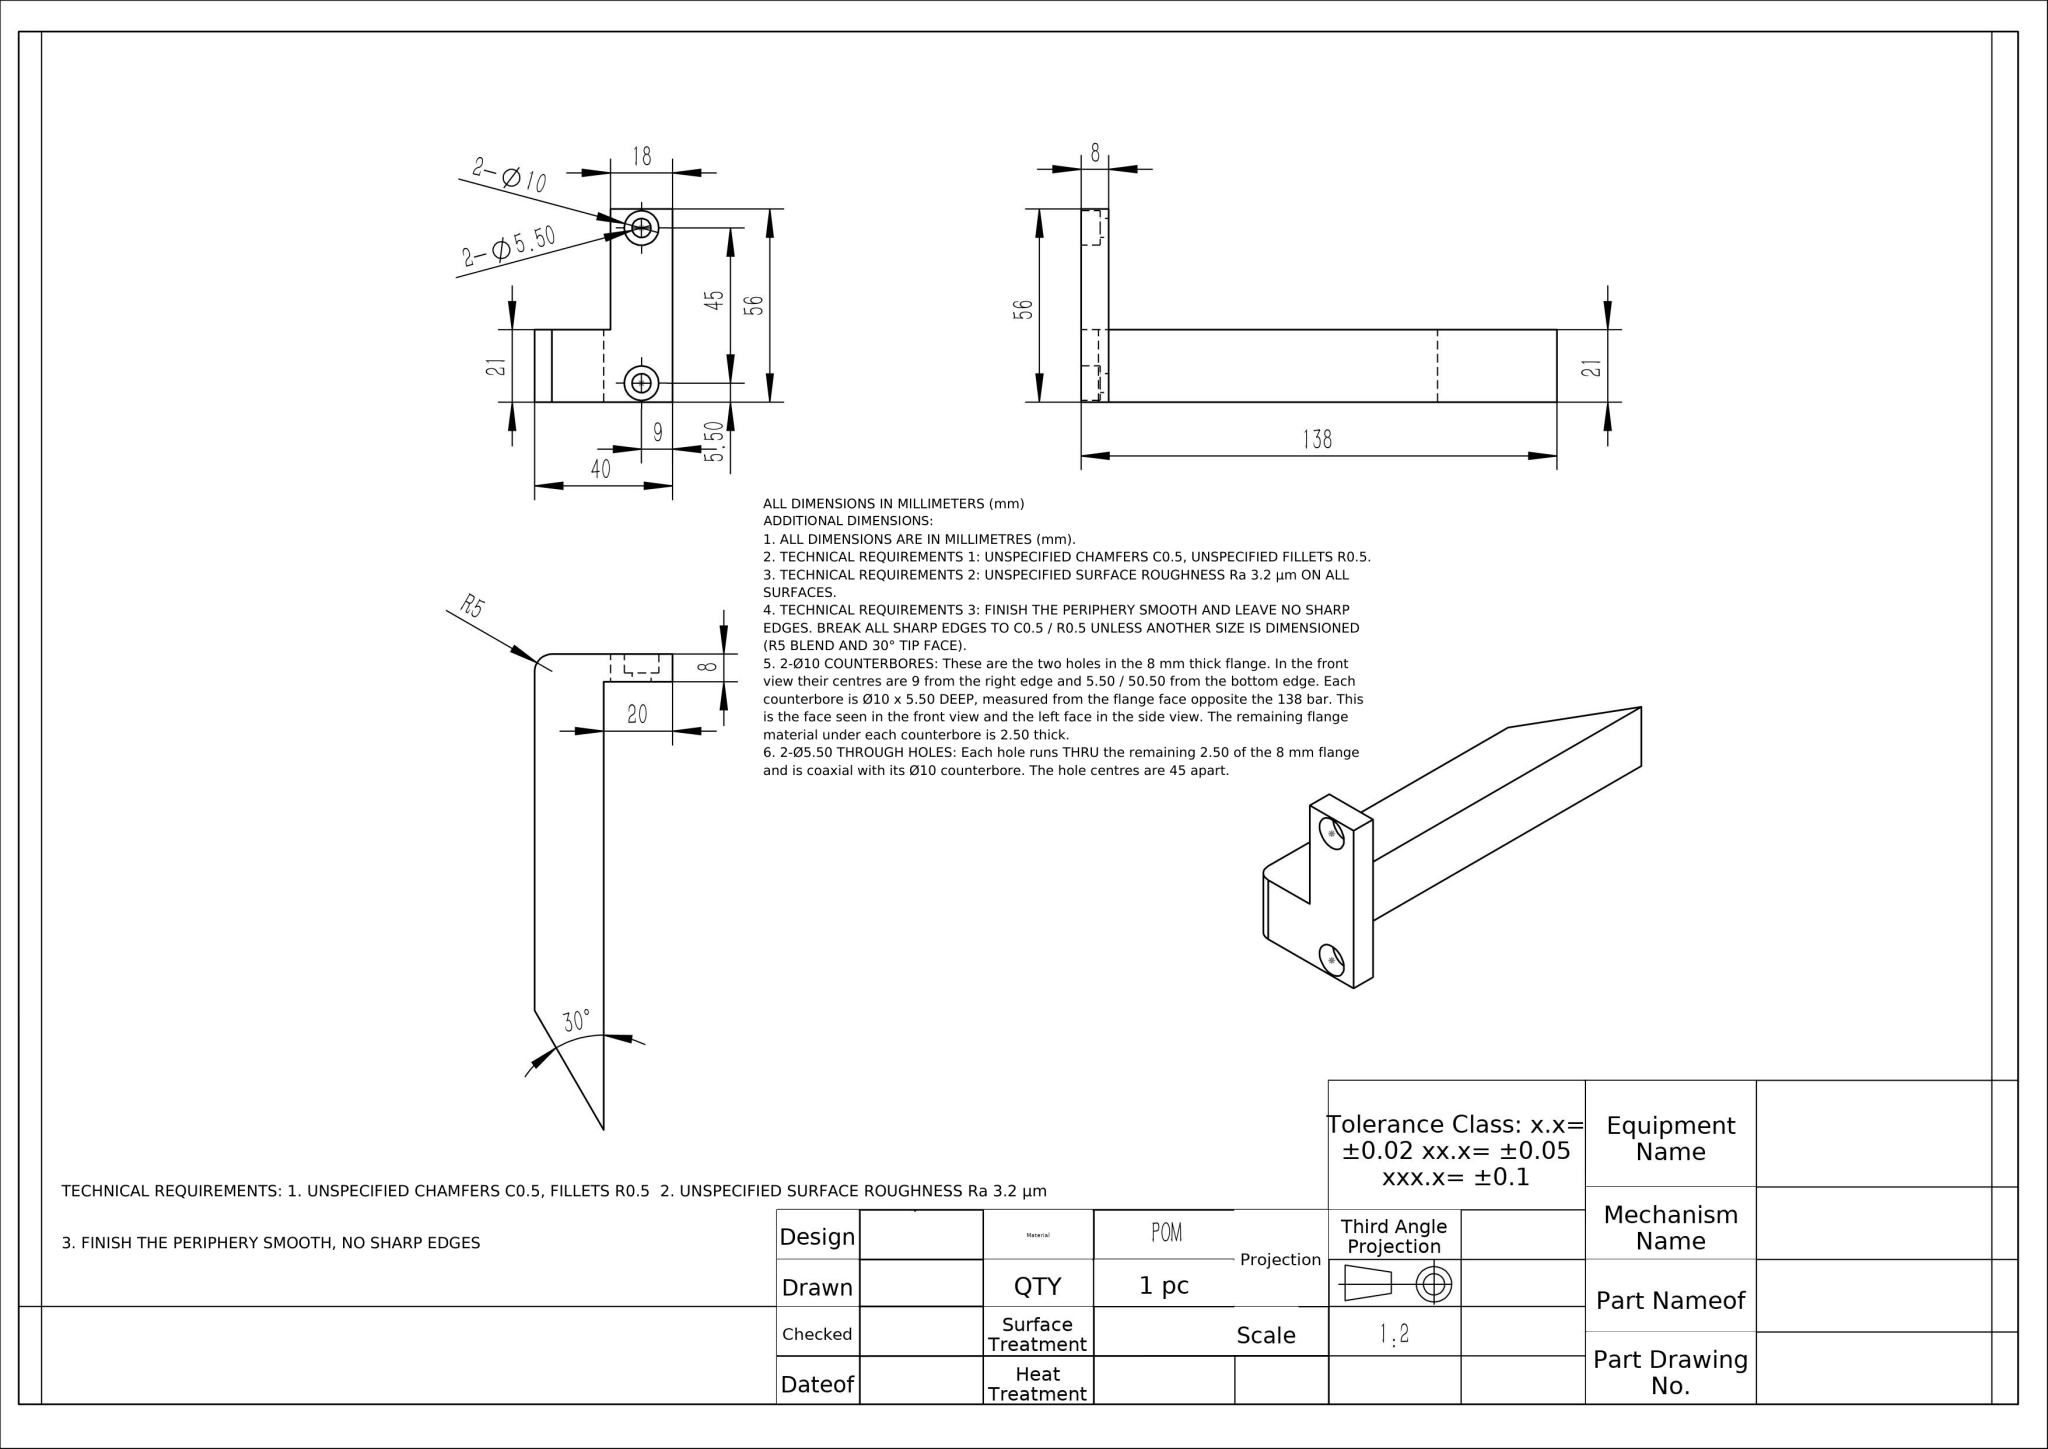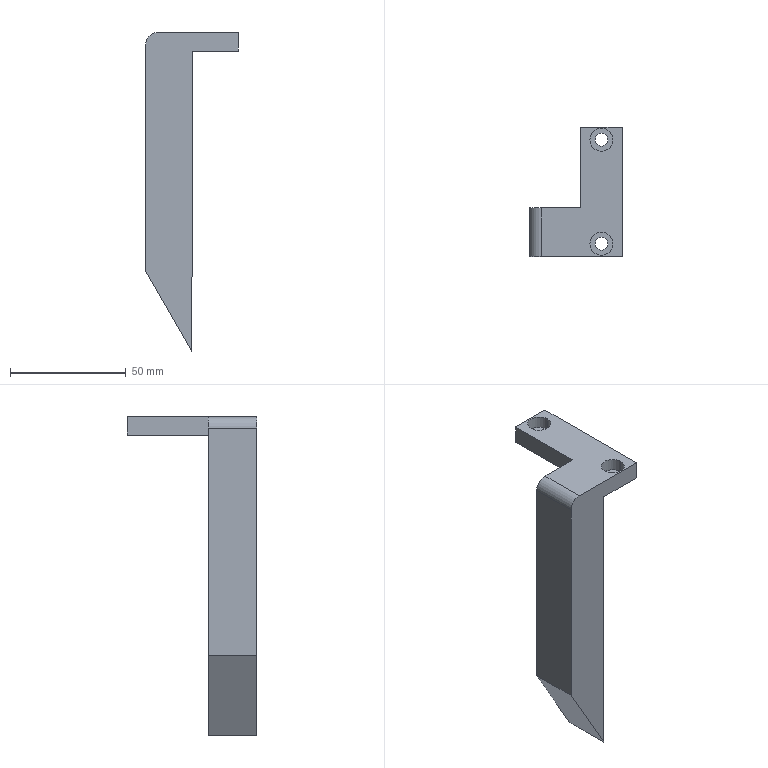Part | NX | mm | Tall L-Shaped Post Bracket | 1 solid | 21 faces | box 40 x 56 x 138 mm | volume 57990 mm3 | plane 12 | cylinder 9 | commonest cylinder face diameters 10 x5 5.5 x4
STEP:
#1=COLOUR_RGB('',0.7922,0.8196,0.9333);
#2=FILL_AREA_STYLE_COLOUR('',#1);
#3=FILL_AREA_STYLE('',(#2));
#4=SURFACE_STYLE_FILL_AREA(#3);
#5=SURFACE_SIDE_STYLE('',(#4));
#6=SURFACE_STYLE_USAGE(.BOTH.,#5);
#7=PRESENTATION_STYLE_ASSIGNMENT((#6));
#8=CARTESIAN_POINT('',(26.,50.5,2.5));
#9=VERTEX_POINT('',#8);
#10=CARTESIAN_POINT('',(36.,50.5,2.5));
#11=VERTEX_POINT('',#10);
#12=CARTESIAN_POINT('',(31.,50.5,2.5));
#13=DIRECTION('',(0.,0.,1.));
#14=DIRECTION('',(1.,0.,0.));
#15=AXIS2_PLACEMENT_3D('',#12,#13,#14);
#16=CIRCLE('',#15,5.);
#17=EDGE_CURVE('',#9,#11,#16,.T.);
#18=ORIENTED_EDGE('',*,*,#17,.F.);
#19=CARTESIAN_POINT('',(26.,50.5,8.));
#20=VERTEX_POINT('',#19);
#21=CARTESIAN_POINT('',(26.,50.5,8.));
#22=DIRECTION('',(0.,0.,1.));
#23=VECTOR('',#22,1000.);
#24=LINE('',#21,#23);
#25=EDGE_CURVE('',#9,#20,#24,.T.);
#26=ORIENTED_EDGE('',*,*,#25,.T.);
#27=CARTESIAN_POINT('',(36.,50.5,8.));
#28=VERTEX_POINT('',#27);
#29=CARTESIAN_POINT('',(31.,50.5,8.));
#30=DIRECTION('',(0.,0.,1.));
#31=DIRECTION('',(1.,0.,0.));
#32=AXIS2_PLACEMENT_3D('',#29,#30,#31);
#33=CIRCLE('',#32,5.);
#34=EDGE_CURVE('',#20,#28,#33,.T.);
#35=ORIENTED_EDGE('',*,*,#34,.T.);
#36=CARTESIAN_POINT('',(36.,50.5,8.));
#37=DIRECTION('',(0.,0.,1.));
#38=VECTOR('',#37,1000.);
#39=LINE('',#36,#38);
#40=EDGE_CURVE('',#11,#28,#39,.T.);
#41=ORIENTED_EDGE('',*,*,#40,.F.);
#42=EDGE_LOOP('',(#18,#26,#35,#41));
#43=FACE_OUTER_BOUND('',#42,.T.);
#44=CARTESIAN_POINT('',(31.,50.5,8.));
#45=DIRECTION('',(0.,0.,1.));
#46=DIRECTION('',(1.,0.,0.));
#47=AXIS2_PLACEMENT_3D('',#44,#45,#46);
#48=CYLINDRICAL_SURFACE('',#47,5.);
#49=ADVANCED_FACE('',(#43),#48,.F.);
#50=CARTESIAN_POINT('',(33.75,50.5,0.));
#51=VERTEX_POINT('',#50);
#52=CARTESIAN_POINT('',(28.25,50.5,0.));
#53=VERTEX_POINT('',#52);
#54=CARTESIAN_POINT('',(31.,50.5,0.));
#55=DIRECTION('',(0.,0.,-1.));
#56=DIRECTION('',(-1.,0.,0.));
#57=AXIS2_PLACEMENT_3D('',#54,#55,#56);
#58=CIRCLE('',#57,2.75);
#59=EDGE_CURVE('',#51,#53,#58,.T.);
#60=ORIENTED_EDGE('',*,*,#59,.T.);
#61=CARTESIAN_POINT('',(28.25,50.5,2.5));
#62=VERTEX_POINT('',#61);
#63=CARTESIAN_POINT('',(28.25,50.5,8.));
#64=DIRECTION('',(0.,0.,1.));
#65=VECTOR('',#64,1000.);
#66=LINE('',#63,#65);
#67=EDGE_CURVE('',#53,#62,#66,.T.);
#68=ORIENTED_EDGE('',*,*,#67,.T.);
#69=CARTESIAN_POINT('',(33.75,50.5,2.5));
#70=VERTEX_POINT('',#69);
#71=CARTESIAN_POINT('',(31.,50.5,2.5));
#72=DIRECTION('',(0.,0.,1.));
#73=DIRECTION('',(1.,0.,0.));
#74=AXIS2_PLACEMENT_3D('',#71,#72,#73);
#75=CIRCLE('',#74,2.75);
#76=EDGE_CURVE('',#62,#70,#75,.T.);
#77=ORIENTED_EDGE('',*,*,#76,.T.);
#78=CARTESIAN_POINT('',(33.75,50.5,8.));
#79=DIRECTION('',(0.,0.,1.));
#80=VECTOR('',#79,1000.);
#81=LINE('',#78,#80);
#82=EDGE_CURVE('',#51,#70,#81,.T.);
#83=ORIENTED_EDGE('',*,*,#82,.F.);
#84=EDGE_LOOP('',(#60,#68,#77,#83));
#85=FACE_OUTER_BOUND('',#84,.T.);
#86=CARTESIAN_POINT('',(31.,50.5,8.));
#87=DIRECTION('',(0.,0.,1.));
#88=DIRECTION('',(1.,0.,0.));
#89=AXIS2_PLACEMENT_3D('',#86,#87,#88);
#90=CYLINDRICAL_SURFACE('',#89,2.75);
#91=ADVANCED_FACE('',(#85),#90,.F.);
#92=CARTESIAN_POINT('',(26.,5.5,2.5));
#93=VERTEX_POINT('',#92);
#94=CARTESIAN_POINT('',(36.,5.5,2.5));
#95=VERTEX_POINT('',#94);
#96=CARTESIAN_POINT('',(31.,5.5,2.5));
#97=DIRECTION('',(0.,0.,1.));
#98=DIRECTION('',(1.,0.,0.));
#99=AXIS2_PLACEMENT_3D('',#96,#97,#98);
#100=CIRCLE('',#99,5.);
#101=EDGE_CURVE('',#93,#95,#100,.T.);
#102=ORIENTED_EDGE('',*,*,#101,.F.);
#103=CARTESIAN_POINT('',(26.,5.5,8.));
#104=VERTEX_POINT('',#103);
#105=CARTESIAN_POINT('',(26.,5.5,8.));
#106=DIRECTION('',(0.,0.,1.));
#107=VECTOR('',#106,1000.);
#108=LINE('',#105,#107);
#109=EDGE_CURVE('',#93,#104,#108,.T.);
#110=ORIENTED_EDGE('',*,*,#109,.T.);
#111=CARTESIAN_POINT('',(36.,5.5,8.));
#112=VERTEX_POINT('',#111);
#113=CARTESIAN_POINT('',(31.,5.5,8.));
#114=DIRECTION('',(0.,0.,1.));
#115=DIRECTION('',(1.,0.,0.));
#116=AXIS2_PLACEMENT_3D('',#113,#114,#115);
#117=CIRCLE('',#116,5.);
#118=EDGE_CURVE('',#104,#112,#117,.T.);
#119=ORIENTED_EDGE('',*,*,#118,.T.);
#120=CARTESIAN_POINT('',(36.,5.5,8.));
#121=DIRECTION('',(0.,0.,1.));
#122=VECTOR('',#121,1000.);
#123=LINE('',#120,#122);
#124=EDGE_CURVE('',#95,#112,#123,.T.);
#125=ORIENTED_EDGE('',*,*,#124,.F.);
#126=EDGE_LOOP('',(#102,#110,#119,#125));
#127=FACE_OUTER_BOUND('',#126,.T.);
#128=CARTESIAN_POINT('',(31.,5.5,8.));
#129=DIRECTION('',(0.,0.,1.));
#130=DIRECTION('',(1.,0.,0.));
#131=AXIS2_PLACEMENT_3D('',#128,#129,#130);
#132=CYLINDRICAL_SURFACE('',#131,5.);
#133=ADVANCED_FACE('',(#127),#132,.F.);
#134=CARTESIAN_POINT('',(33.75,5.5,0.));
#135=VERTEX_POINT('',#134);
#136=CARTESIAN_POINT('',(28.25,5.5,0.));
#137=VERTEX_POINT('',#136);
#138=CARTESIAN_POINT('',(31.,5.5,0.));
#139=DIRECTION('',(0.,0.,-1.));
#140=DIRECTION('',(-1.,0.,0.));
#141=AXIS2_PLACEMENT_3D('',#138,#139,#140);
#142=CIRCLE('',#141,2.75);
#143=EDGE_CURVE('',#135,#137,#142,.T.);
#144=ORIENTED_EDGE('',*,*,#143,.T.);
#145=CARTESIAN_POINT('',(28.25,5.5,2.5));
#146=VERTEX_POINT('',#145);
#147=CARTESIAN_POINT('',(28.25,5.5,8.));
#148=DIRECTION('',(0.,0.,1.));
#149=VECTOR('',#148,1000.);
#150=LINE('',#147,#149);
#151=EDGE_CURVE('',#137,#146,#150,.T.);
#152=ORIENTED_EDGE('',*,*,#151,.T.);
#153=CARTESIAN_POINT('',(33.75,5.5,2.5));
#154=VERTEX_POINT('',#153);
#155=CARTESIAN_POINT('',(31.,5.5,2.5));
#156=DIRECTION('',(0.,0.,1.));
#157=DIRECTION('',(1.,0.,0.));
#158=AXIS2_PLACEMENT_3D('',#155,#156,#157);
#159=CIRCLE('',#158,2.75);
#160=EDGE_CURVE('',#146,#154,#159,.T.);
#161=ORIENTED_EDGE('',*,*,#160,.T.);
#162=CARTESIAN_POINT('',(33.75,5.5,8.));
#163=DIRECTION('',(0.,0.,1.));
#164=VECTOR('',#163,1000.);
#165=LINE('',#162,#164);
#166=EDGE_CURVE('',#135,#154,#165,.T.);
#167=ORIENTED_EDGE('',*,*,#166,.F.);
#168=EDGE_LOOP('',(#144,#152,#161,#167));
#169=FACE_OUTER_BOUND('',#168,.T.);
#170=CARTESIAN_POINT('',(31.,5.5,8.));
#171=DIRECTION('',(0.,0.,1.));
#172=DIRECTION('',(1.,0.,0.));
#173=AXIS2_PLACEMENT_3D('',#170,#171,#172);
#174=CYLINDRICAL_SURFACE('',#173,2.75);
#175=ADVANCED_FACE('',(#169),#174,.F.);
#176=ORIENTED_EDGE('',*,*,#59,.F.);
#177=CARTESIAN_POINT('',(31.,50.5,0.));
#178=DIRECTION('',(0.,0.,-1.));
#179=DIRECTION('',(-1.,0.,0.));
#180=AXIS2_PLACEMENT_3D('',#177,#178,#179);
#181=CIRCLE('',#180,2.75);
#182=EDGE_CURVE('',#53,#51,#181,.T.);
#183=ORIENTED_EDGE('',*,*,#182,.F.);
#184=EDGE_LOOP('',(#176,#183));
#185=FACE_BOUND('',#184,.T.);
#186=ORIENTED_EDGE('',*,*,#143,.F.);
#187=CARTESIAN_POINT('',(31.,5.5,0.));
#188=DIRECTION('',(0.,0.,-1.));
#189=DIRECTION('',(-1.,0.,0.));
#190=AXIS2_PLACEMENT_3D('',#187,#188,#189);
#191=CIRCLE('',#190,2.75);
#192=EDGE_CURVE('',#137,#135,#191,.T.);
#193=ORIENTED_EDGE('',*,*,#192,.F.);
#194=EDGE_LOOP('',(#186,#193));
#195=FACE_BOUND('',#194,.T.);
#196=CARTESIAN_POINT('',(20.,0.,0.));
#197=VERTEX_POINT('',#196);
#198=CARTESIAN_POINT('',(40.,0.,0.));
#199=VERTEX_POINT('',#198);
#200=CARTESIAN_POINT('',(0.,0.,0.));
#201=DIRECTION('',(1.,0.,0.));
#202=VECTOR('',#201,1000.);
#203=LINE('',#200,#202);
#204=EDGE_CURVE('',#197,#199,#203,.T.);
#205=ORIENTED_EDGE('',*,*,#204,.F.);
#206=CARTESIAN_POINT('',(20.,21.,0.));
#207=VERTEX_POINT('',#206);
#208=CARTESIAN_POINT('',(20.,-131.529,0.));
#209=DIRECTION('',(-0.,1.,0.));
#210=VECTOR('',#209,1000.);
#211=LINE('',#208,#210);
#212=EDGE_CURVE('',#197,#207,#211,.T.);
#213=ORIENTED_EDGE('',*,*,#212,.T.);
#214=CARTESIAN_POINT('',(22.,21.,0.));
#215=VERTEX_POINT('',#214);
#216=CARTESIAN_POINT('',(0.,21.,0.));
#217=DIRECTION('',(1.,0.,0.));
#218=VECTOR('',#217,1000.);
#219=LINE('',#216,#218);
#220=EDGE_CURVE('',#207,#215,#219,.T.);
#221=ORIENTED_EDGE('',*,*,#220,.T.);
#222=CARTESIAN_POINT('',(22.,56.,0.));
#223=VERTEX_POINT('',#222);
#224=CARTESIAN_POINT('',(22.,56.,0.));
#225=DIRECTION('',(-0.,1.,0.));
#226=VECTOR('',#225,1000.);
#227=LINE('',#224,#226);
#228=EDGE_CURVE('',#215,#223,#227,.T.);
#229=ORIENTED_EDGE('',*,*,#228,.T.);
#230=CARTESIAN_POINT('',(40.,56.,0.));
#231=VERTEX_POINT('',#230);
#232=CARTESIAN_POINT('',(0.,56.,0.));
#233=DIRECTION('',(-1.,0.,0.));
#234=VECTOR('',#233,1000.);
#235=LINE('',#232,#234);
#236=EDGE_CURVE('',#231,#223,#235,.T.);
#237=ORIENTED_EDGE('',*,*,#236,.F.);
#238=CARTESIAN_POINT('',(40.,0.,0.));
#239=DIRECTION('',(0.,1.,0.));
#240=VECTOR('',#239,1000.);
#241=LINE('',#238,#240);
#242=EDGE_CURVE('',#199,#231,#241,.T.);
#243=ORIENTED_EDGE('',*,*,#242,.F.);
#244=EDGE_LOOP('',(#205,#213,#221,#229,#237,#243));
#245=FACE_OUTER_BOUND('',#244,.T.);
#246=CARTESIAN_POINT('',(0.,0.,0.));
#247=DIRECTION('',(0.,0.,-1.));
#248=DIRECTION('',(-1.,0.,0.));
#249=AXIS2_PLACEMENT_3D('',#246,#247,#248);
#250=PLANE('',#249);
#251=ADVANCED_FACE('',(#185,#195,#245),#250,.T.);
#252=CARTESIAN_POINT('',(0.,0.,3.));
#253=VERTEX_POINT('',#252);
#254=CARTESIAN_POINT('',(0.,0.,-95.359));
#255=VERTEX_POINT('',#254);
#256=CARTESIAN_POINT('',(0.,0.,8.));
#257=DIRECTION('',(0.,0.,-1.));
#258=VECTOR('',#257,1000.);
#259=LINE('',#256,#258);
#260=EDGE_CURVE('',#253,#255,#259,.T.);
#261=ORIENTED_EDGE('',*,*,#260,.F.);
#262=CARTESIAN_POINT('',(0.,21.,3.));
#263=VERTEX_POINT('',#262);
#264=CARTESIAN_POINT('',(0.,0.,3.));
#265=DIRECTION('',(0.,1.,0.));
#266=VECTOR('',#265,1000.);
#267=LINE('',#264,#266);
#268=EDGE_CURVE('',#253,#263,#267,.T.);
#269=ORIENTED_EDGE('',*,*,#268,.T.);
#270=CARTESIAN_POINT('',(0.,21.,-95.359));
#271=VERTEX_POINT('',#270);
#272=CARTESIAN_POINT('',(0.,21.,0.));
#273=DIRECTION('',(0.,0.,1.));
#274=VECTOR('',#273,1000.);
#275=LINE('',#272,#274);
#276=EDGE_CURVE('',#271,#263,#275,.T.);
#277=ORIENTED_EDGE('',*,*,#276,.F.);
#278=CARTESIAN_POINT('',(0.,-131.529,-95.359));
#279=DIRECTION('',(-0.,1.,0.));
#280=VECTOR('',#279,1000.);
#281=LINE('',#278,#280);
#282=EDGE_CURVE('',#255,#271,#281,.T.);
#283=ORIENTED_EDGE('',*,*,#282,.F.);
#284=EDGE_LOOP('',(#261,#269,#277,#283));
#285=FACE_OUTER_BOUND('',#284,.T.);
#286=CARTESIAN_POINT('',(0.,0.,8.));
#287=DIRECTION('',(1.,0.,0.));
#288=DIRECTION('',(0.,0.,-1.));
#289=AXIS2_PLACEMENT_3D('',#286,#287,#288);
#290=PLANE('',#289);
#291=ADVANCED_FACE('',(#285),#290,.F.);
#292=CARTESIAN_POINT('',(5.,0.,8.));
#293=VERTEX_POINT('',#292);
#294=CARTESIAN_POINT('',(40.,0.,8.));
#295=VERTEX_POINT('',#294);
#296=CARTESIAN_POINT('',(0.,0.,8.));
#297=DIRECTION('',(1.,0.,0.));
#298=VECTOR('',#297,1000.);
#299=LINE('',#296,#298);
#300=EDGE_CURVE('',#293,#295,#299,.T.);
#301=ORIENTED_EDGE('',*,*,#300,.F.);
#302=CARTESIAN_POINT('',(5.,0.,3.));
#303=DIRECTION('',(0.,-1.,0.));
#304=DIRECTION('',(0.,0.,1.));
#305=AXIS2_PLACEMENT_3D('',#302,#303,#304);
#306=CIRCLE('',#305,5.);
#307=EDGE_CURVE('',#293,#253,#306,.T.);
#308=ORIENTED_EDGE('',*,*,#307,.T.);
#309=ORIENTED_EDGE('',*,*,#260,.T.);
#310=CARTESIAN_POINT('',(20.,0.,-130.));
#311=VERTEX_POINT('',#310);
#312=CARTESIAN_POINT('',(0.,0.,-95.359));
#313=DIRECTION('',(0.5,0.,-0.866));
#314=VECTOR('',#313,1000.);
#315=LINE('',#312,#314);
#316=EDGE_CURVE('',#255,#311,#315,.T.);
#317=ORIENTED_EDGE('',*,*,#316,.T.);
#318=CARTESIAN_POINT('',(20.,0.,-130.));
#319=DIRECTION('',(0.,0.,1.));
#320=VECTOR('',#319,1000.);
#321=LINE('',#318,#320);
#322=EDGE_CURVE('',#311,#197,#321,.T.);
#323=ORIENTED_EDGE('',*,*,#322,.T.);
#324=ORIENTED_EDGE('',*,*,#204,.T.);
#325=CARTESIAN_POINT('',(40.,0.,8.));
#326=DIRECTION('',(0.,0.,-1.));
#327=VECTOR('',#326,1000.);
#328=LINE('',#325,#327);
#329=EDGE_CURVE('',#295,#199,#328,.T.);
#330=ORIENTED_EDGE('',*,*,#329,.F.);
#331=EDGE_LOOP('',(#301,#308,#309,#317,#323,#324,#330));
#332=FACE_OUTER_BOUND('',#331,.T.);
#333=CARTESIAN_POINT('',(0.,0.,8.));
#334=DIRECTION('',(0.,1.,0.));
#335=DIRECTION('',(0.,0.,1.));
#336=AXIS2_PLACEMENT_3D('',#333,#334,#335);
#337=PLANE('',#336);
#338=ADVANCED_FACE('',(#332),#337,.F.);
#339=ORIENTED_EDGE('',*,*,#242,.T.);
#340=CARTESIAN_POINT('',(40.,56.,8.));
#341=VERTEX_POINT('',#340);
#342=CARTESIAN_POINT('',(40.,56.,8.));
#343=DIRECTION('',(0.,0.,-1.));
#344=VECTOR('',#343,1000.);
#345=LINE('',#342,#344);
#346=EDGE_CURVE('',#341,#231,#345,.T.);
#347=ORIENTED_EDGE('',*,*,#346,.F.);
#348=CARTESIAN_POINT('',(40.,0.,8.));
#349=DIRECTION('',(0.,1.,0.));
#350=VECTOR('',#349,1000.);
#351=LINE('',#348,#350);
#352=EDGE_CURVE('',#295,#341,#351,.T.);
#353=ORIENTED_EDGE('',*,*,#352,.F.);
#354=ORIENTED_EDGE('',*,*,#329,.T.);
#355=EDGE_LOOP('',(#339,#347,#353,#354));
#356=FACE_OUTER_BOUND('',#355,.T.);
#357=CARTESIAN_POINT('',(40.,0.,8.));
#358=DIRECTION('',(-1.,0.,0.));
#359=DIRECTION('',(0.,0.,1.));
#360=AXIS2_PLACEMENT_3D('',#357,#358,#359);
#361=PLANE('',#360);
#362=ADVANCED_FACE('',(#356),#361,.F.);
#363=ORIENTED_EDGE('',*,*,#236,.T.);
#364=CARTESIAN_POINT('',(22.,56.,8.));
#365=VERTEX_POINT('',#364);
#366=CARTESIAN_POINT('',(22.,56.,0.));
#367=DIRECTION('',(0.,0.,1.));
#368=VECTOR('',#367,1000.);
#369=LINE('',#366,#368);
#370=EDGE_CURVE('',#223,#365,#369,.T.);
#371=ORIENTED_EDGE('',*,*,#370,.T.);
#372=CARTESIAN_POINT('',(0.,56.,8.));
#373=DIRECTION('',(-1.,0.,0.));
#374=VECTOR('',#373,1000.);
#375=LINE('',#372,#374);
#376=EDGE_CURVE('',#341,#365,#375,.T.);
#377=ORIENTED_EDGE('',*,*,#376,.F.);
#378=ORIENTED_EDGE('',*,*,#346,.T.);
#379=EDGE_LOOP('',(#363,#371,#377,#378));
#380=FACE_OUTER_BOUND('',#379,.T.);
#381=CARTESIAN_POINT('',(0.,56.,8.));
#382=DIRECTION('',(0.,-1.,0.));
#383=DIRECTION('',(0.,0.,-1.));
#384=AXIS2_PLACEMENT_3D('',#381,#382,#383);
#385=PLANE('',#384);
#386=ADVANCED_FACE('',(#380),#385,.F.);
#387=CARTESIAN_POINT('',(31.,50.5,8.));
#388=DIRECTION('',(0.,0.,1.));
#389=DIRECTION('',(1.,0.,0.));
#390=AXIS2_PLACEMENT_3D('',#387,#388,#389);
#391=CIRCLE('',#390,5.);
#392=EDGE_CURVE('',#28,#20,#391,.T.);
#393=ORIENTED_EDGE('',*,*,#392,.F.);
#394=ORIENTED_EDGE('',*,*,#34,.F.);
#395=EDGE_LOOP('',(#393,#394));
#396=FACE_BOUND('',#395,.T.);
#397=CARTESIAN_POINT('',(31.,5.5,8.));
#398=DIRECTION('',(0.,0.,1.));
#399=DIRECTION('',(1.,0.,0.));
#400=AXIS2_PLACEMENT_3D('',#397,#398,#399);
#401=CIRCLE('',#400,5.);
#402=EDGE_CURVE('',#112,#104,#401,.T.);
#403=ORIENTED_EDGE('',*,*,#402,.F.);
#404=ORIENTED_EDGE('',*,*,#118,.F.);
#405=EDGE_LOOP('',(#403,#404));
#406=FACE_BOUND('',#405,.T.);
#407=CARTESIAN_POINT('',(5.,21.,8.));
#408=VERTEX_POINT('',#407);
#409=CARTESIAN_POINT('',(22.,21.,8.));
#410=VERTEX_POINT('',#409);
#411=CARTESIAN_POINT('',(0.,21.,8.));
#412=DIRECTION('',(1.,0.,0.));
#413=VECTOR('',#412,1000.);
#414=LINE('',#411,#413);
#415=EDGE_CURVE('',#408,#410,#414,.T.);
#416=ORIENTED_EDGE('',*,*,#415,.F.);
#417=CARTESIAN_POINT('',(5.,0.,8.));
#418=DIRECTION('',(0.,-1.,0.));
#419=VECTOR('',#418,1000.);
#420=LINE('',#417,#419);
#421=EDGE_CURVE('',#408,#293,#420,.T.);
#422=ORIENTED_EDGE('',*,*,#421,.T.);
#423=ORIENTED_EDGE('',*,*,#300,.T.);
#424=ORIENTED_EDGE('',*,*,#352,.T.);
#425=ORIENTED_EDGE('',*,*,#376,.T.);
#426=CARTESIAN_POINT('',(22.,56.,8.));
#427=DIRECTION('',(-0.,1.,0.));
#428=VECTOR('',#427,1000.);
#429=LINE('',#426,#428);
#430=EDGE_CURVE('',#410,#365,#429,.T.);
#431=ORIENTED_EDGE('',*,*,#430,.F.);
#432=EDGE_LOOP('',(#416,#422,#423,#424,#425,#431));
#433=FACE_OUTER_BOUND('',#432,.T.);
#434=CARTESIAN_POINT('',(0.,0.,8.));
#435=DIRECTION('',(0.,0.,-1.));
#436=DIRECTION('',(-1.,0.,0.));
#437=AXIS2_PLACEMENT_3D('',#434,#435,#436);
#438=PLANE('',#437);
#439=ADVANCED_FACE('',(#396,#406,#433),#438,.F.);
#440=ORIENTED_EDGE('',*,*,#430,.T.);
#441=ORIENTED_EDGE('',*,*,#370,.F.);
#442=ORIENTED_EDGE('',*,*,#228,.F.);
#443=CARTESIAN_POINT('',(22.,21.,0.));
#444=DIRECTION('',(0.,0.,1.));
#445=VECTOR('',#444,1000.);
#446=LINE('',#443,#445);
#447=EDGE_CURVE('',#215,#410,#446,.T.);
#448=ORIENTED_EDGE('',*,*,#447,.T.);
#449=EDGE_LOOP('',(#440,#441,#442,#448));
#450=FACE_OUTER_BOUND('',#449,.T.);
#451=CARTESIAN_POINT('',(22.,56.,0.));
#452=DIRECTION('',(1.,0.,0.));
#453=DIRECTION('',(-0.,1.,0.));
#454=AXIS2_PLACEMENT_3D('',#451,#452,#453);
#455=PLANE('',#454);
#456=ADVANCED_FACE('',(#450),#455,.F.);
#457=ORIENTED_EDGE('',*,*,#276,.T.);
#458=CARTESIAN_POINT('',(5.,21.,3.));
#459=DIRECTION('',(0.,1.,0.));
#460=DIRECTION('',(0.,0.,-1.));
#461=AXIS2_PLACEMENT_3D('',#458,#459,#460);
#462=CIRCLE('',#461,5.);
#463=EDGE_CURVE('',#263,#408,#462,.T.);
#464=ORIENTED_EDGE('',*,*,#463,.T.);
#465=ORIENTED_EDGE('',*,*,#415,.T.);
#466=ORIENTED_EDGE('',*,*,#447,.F.);
#467=ORIENTED_EDGE('',*,*,#220,.F.);
#468=CARTESIAN_POINT('',(20.,21.,-130.));
#469=VERTEX_POINT('',#468);
#470=CARTESIAN_POINT('',(20.,21.,-130.));
#471=DIRECTION('',(-0.,0.,-1.));
#472=VECTOR('',#471,1000.);
#473=LINE('',#470,#472);
#474=EDGE_CURVE('',#207,#469,#473,.T.);
#475=ORIENTED_EDGE('',*,*,#474,.T.);
#476=CARTESIAN_POINT('',(0.,21.,-95.359));
#477=DIRECTION('',(-0.5,-0.,0.866));
#478=VECTOR('',#477,1000.);
#479=LINE('',#476,#478);
#480=EDGE_CURVE('',#469,#271,#479,.T.);
#481=ORIENTED_EDGE('',*,*,#480,.T.);
#482=EDGE_LOOP('',(#457,#464,#465,#466,#467,#475,#481));
#483=FACE_OUTER_BOUND('',#482,.T.);
#484=CARTESIAN_POINT('',(0.,21.,0.));
#485=DIRECTION('',(0.,-1.,0.));
#486=DIRECTION('',(0.,0.,-1.));
#487=AXIS2_PLACEMENT_3D('',#484,#485,#486);
#488=PLANE('',#487);
#489=ADVANCED_FACE('',(#483),#488,.F.);
#490=ORIENTED_EDGE('',*,*,#316,.F.);
#491=ORIENTED_EDGE('',*,*,#282,.T.);
#492=ORIENTED_EDGE('',*,*,#480,.F.);
#493=CARTESIAN_POINT('',(20.,-131.529,-130.));
#494=DIRECTION('',(-0.,1.,0.));
#495=VECTOR('',#494,1000.);
#496=LINE('',#493,#495);
#497=EDGE_CURVE('',#311,#469,#496,.T.);
#498=ORIENTED_EDGE('',*,*,#497,.F.);
#499=EDGE_LOOP('',(#490,#491,#492,#498));
#500=FACE_OUTER_BOUND('',#499,.T.);
#501=CARTESIAN_POINT('',(0.,-131.529,-95.359));
#502=DIRECTION('',(-0.866,-0.,-0.5));
#503=DIRECTION('',(-0.5,0.,0.866));
#504=AXIS2_PLACEMENT_3D('',#501,#502,#503);
#505=PLANE('',#504);
#506=ADVANCED_FACE('',(#500),#505,.T.);
#507=ORIENTED_EDGE('',*,*,#322,.F.);
#508=ORIENTED_EDGE('',*,*,#497,.T.);
#509=ORIENTED_EDGE('',*,*,#474,.F.);
#510=ORIENTED_EDGE('',*,*,#212,.F.);
#511=EDGE_LOOP('',(#507,#508,#509,#510));
#512=FACE_OUTER_BOUND('',#511,.T.);
#513=CARTESIAN_POINT('',(20.,-131.529,-130.));
#514=DIRECTION('',(1.,0.,-0.));
#515=DIRECTION('',(-0.,0.,-1.));
#516=AXIS2_PLACEMENT_3D('',#513,#514,#515);
#517=PLANE('',#516);
#518=ADVANCED_FACE('',(#512),#517,.T.);
#519=ORIENTED_EDGE('',*,*,#151,.F.);
#520=ORIENTED_EDGE('',*,*,#192,.T.);
#521=ORIENTED_EDGE('',*,*,#166,.T.);
#522=CARTESIAN_POINT('',(31.,5.5,2.5));
#523=DIRECTION('',(0.,0.,1.));
#524=DIRECTION('',(1.,0.,0.));
#525=AXIS2_PLACEMENT_3D('',#522,#523,#524);
#526=CIRCLE('',#525,2.75);
#527=EDGE_CURVE('',#154,#146,#526,.T.);
#528=ORIENTED_EDGE('',*,*,#527,.T.);
#529=EDGE_LOOP('',(#519,#520,#521,#528));
#530=FACE_OUTER_BOUND('',#529,.T.);
#531=CARTESIAN_POINT('',(31.,5.5,8.));
#532=DIRECTION('',(0.,0.,1.));
#533=DIRECTION('',(1.,0.,0.));
#534=AXIS2_PLACEMENT_3D('',#531,#532,#533);
#535=CYLINDRICAL_SURFACE('',#534,2.75);
#536=ADVANCED_FACE('',(#530),#535,.F.);
#537=ORIENTED_EDGE('',*,*,#527,.F.);
#538=ORIENTED_EDGE('',*,*,#160,.F.);
#539=EDGE_LOOP('',(#537,#538));
#540=FACE_BOUND('',#539,.T.);
#541=CARTESIAN_POINT('',(31.,5.5,2.5));
#542=DIRECTION('',(0.,0.,1.));
#543=DIRECTION('',(1.,0.,0.));
#544=AXIS2_PLACEMENT_3D('',#541,#542,#543);
#545=CIRCLE('',#544,5.);
#546=EDGE_CURVE('',#95,#93,#545,.T.);
#547=ORIENTED_EDGE('',*,*,#546,.T.);
#548=ORIENTED_EDGE('',*,*,#101,.T.);
#549=EDGE_LOOP('',(#547,#548));
#550=FACE_OUTER_BOUND('',#549,.T.);
#551=CARTESIAN_POINT('',(33.75,5.5,2.5));
#552=DIRECTION('',(0.,0.,-1.));
#553=DIRECTION('',(-1.,0.,0.));
#554=AXIS2_PLACEMENT_3D('',#551,#552,#553);
#555=PLANE('',#554);
#556=ADVANCED_FACE('',(#540,#550),#555,.F.);
#557=ORIENTED_EDGE('',*,*,#109,.F.);
#558=ORIENTED_EDGE('',*,*,#546,.F.);
#559=ORIENTED_EDGE('',*,*,#124,.T.);
#560=ORIENTED_EDGE('',*,*,#402,.T.);
#561=EDGE_LOOP('',(#557,#558,#559,#560));
#562=FACE_OUTER_BOUND('',#561,.T.);
#563=CARTESIAN_POINT('',(31.,5.5,8.));
#564=DIRECTION('',(0.,0.,1.));
#565=DIRECTION('',(1.,0.,0.));
#566=AXIS2_PLACEMENT_3D('',#563,#564,#565);
#567=CYLINDRICAL_SURFACE('',#566,5.);
#568=ADVANCED_FACE('',(#562),#567,.F.);
#569=ORIENTED_EDGE('',*,*,#67,.F.);
#570=ORIENTED_EDGE('',*,*,#182,.T.);
#571=ORIENTED_EDGE('',*,*,#82,.T.);
#572=CARTESIAN_POINT('',(31.,50.5,2.5));
#573=DIRECTION('',(0.,0.,1.));
#574=DIRECTION('',(1.,0.,0.));
#575=AXIS2_PLACEMENT_3D('',#572,#573,#574);
#576=CIRCLE('',#575,2.75);
#577=EDGE_CURVE('',#70,#62,#576,.T.);
#578=ORIENTED_EDGE('',*,*,#577,.T.);
#579=EDGE_LOOP('',(#569,#570,#571,#578));
#580=FACE_OUTER_BOUND('',#579,.T.);
#581=CARTESIAN_POINT('',(31.,50.5,8.));
#582=DIRECTION('',(0.,0.,1.));
#583=DIRECTION('',(1.,0.,0.));
#584=AXIS2_PLACEMENT_3D('',#581,#582,#583);
#585=CYLINDRICAL_SURFACE('',#584,2.75);
#586=ADVANCED_FACE('',(#580),#585,.F.);
#587=ORIENTED_EDGE('',*,*,#577,.F.);
#588=ORIENTED_EDGE('',*,*,#76,.F.);
#589=EDGE_LOOP('',(#587,#588));
#590=FACE_BOUND('',#589,.T.);
#591=CARTESIAN_POINT('',(31.,50.5,2.5));
#592=DIRECTION('',(0.,0.,1.));
#593=DIRECTION('',(1.,0.,0.));
#594=AXIS2_PLACEMENT_3D('',#591,#592,#593);
#595=CIRCLE('',#594,5.);
#596=EDGE_CURVE('',#11,#9,#595,.T.);
#597=ORIENTED_EDGE('',*,*,#596,.T.);
#598=ORIENTED_EDGE('',*,*,#17,.T.);
#599=EDGE_LOOP('',(#597,#598));
#600=FACE_OUTER_BOUND('',#599,.T.);
#601=CARTESIAN_POINT('',(33.75,50.5,2.5));
#602=DIRECTION('',(0.,0.,-1.));
#603=DIRECTION('',(-1.,0.,0.));
#604=AXIS2_PLACEMENT_3D('',#601,#602,#603);
#605=PLANE('',#604);
#606=ADVANCED_FACE('',(#590,#600),#605,.F.);
#607=ORIENTED_EDGE('',*,*,#25,.F.);
#608=ORIENTED_EDGE('',*,*,#596,.F.);
#609=ORIENTED_EDGE('',*,*,#40,.T.);
#610=ORIENTED_EDGE('',*,*,#392,.T.);
#611=EDGE_LOOP('',(#607,#608,#609,#610));
#612=FACE_OUTER_BOUND('',#611,.T.);
#613=CARTESIAN_POINT('',(31.,50.5,8.));
#614=DIRECTION('',(0.,0.,1.));
#615=DIRECTION('',(1.,0.,0.));
#616=AXIS2_PLACEMENT_3D('',#613,#614,#615);
#617=CYLINDRICAL_SURFACE('',#616,5.);
#618=ADVANCED_FACE('',(#612),#617,.F.);
#619=ORIENTED_EDGE('',*,*,#463,.F.);
#620=ORIENTED_EDGE('',*,*,#268,.F.);
#621=ORIENTED_EDGE('',*,*,#307,.F.);
#622=ORIENTED_EDGE('',*,*,#421,.F.);
#623=EDGE_LOOP('',(#619,#620,#621,#622));
#624=FACE_OUTER_BOUND('',#623,.T.);
#625=CARTESIAN_POINT('',(5.,0.,3.));
#626=DIRECTION('',(0.,-1.,0.));
#627=DIRECTION('',(0.,0.,-1.));
#628=AXIS2_PLACEMENT_3D('',#625,#626,#627);
#629=CYLINDRICAL_SURFACE('',#628,5.);
#630=ADVANCED_FACE('',(#624),#629,.T.);
#631=CLOSED_SHELL('',(#49,#91,#133,#175,#251,#291,#338,#362,#386,#439,#456,#489,#506,#518,#536,#556,#568,#586,#606,#618,#630));
#632=MANIFOLD_SOLID_BREP('',#631);
#633=STYLED_ITEM('',(#7),#632);
#634=(LENGTH_UNIT()NAMED_UNIT(*)SI_UNIT(.MILLI.,.METRE.));
#635=UNCERTAINTY_MEASURE_WITH_UNIT(LENGTH_MEASURE(0.00001),#634,'','');
#636=(NAMED_UNIT(*)PLANE_ANGLE_UNIT()SI_UNIT($,.RADIAN.));
#637=(NAMED_UNIT(*)SI_UNIT($,.STERADIAN.)SOLID_ANGLE_UNIT());
#638=(GEOMETRIC_REPRESENTATION_CONTEXT(3)GLOBAL_UNCERTAINTY_ASSIGNED_CONTEXT((#635))GLOBAL_UNIT_ASSIGNED_CONTEXT((#634,#636,#637))REPRESENTATION_CONTEXT('',''));
#639=MECHANICAL_DESIGN_GEOMETRIC_PRESENTATION_REPRESENTATION('',(#633),#638);
#640=CARTESIAN_POINT('',(0.,0.,0.));
#641=DIRECTION('',(0.,0.,1.));
#642=DIRECTION('',(1.,0.,0.));
#643=AXIS2_PLACEMENT_3D('',#640,#641,#642);
#644=(LENGTH_UNIT()NAMED_UNIT(*)SI_UNIT(.MILLI.,.METRE.));
#645=UNCERTAINTY_MEASURE_WITH_UNIT(LENGTH_MEASURE(0.00001),#644,'','');
#646=(NAMED_UNIT(*)PLANE_ANGLE_UNIT()SI_UNIT($,.RADIAN.));
#647=(NAMED_UNIT(*)SI_UNIT($,.STERADIAN.)SOLID_ANGLE_UNIT());
#648=(GEOMETRIC_REPRESENTATION_CONTEXT(3)GLOBAL_UNCERTAINTY_ASSIGNED_CONTEXT((#645))GLOBAL_UNIT_ASSIGNED_CONTEXT((#644,#646,#647))REPRESENTATION_CONTEXT('',''));
#649=ADVANCED_BREP_SHAPE_REPRESENTATION('',(#632,#643),#648);
#650=PRESENTATION_LAYER_ASSIGNMENT('','',(#633));